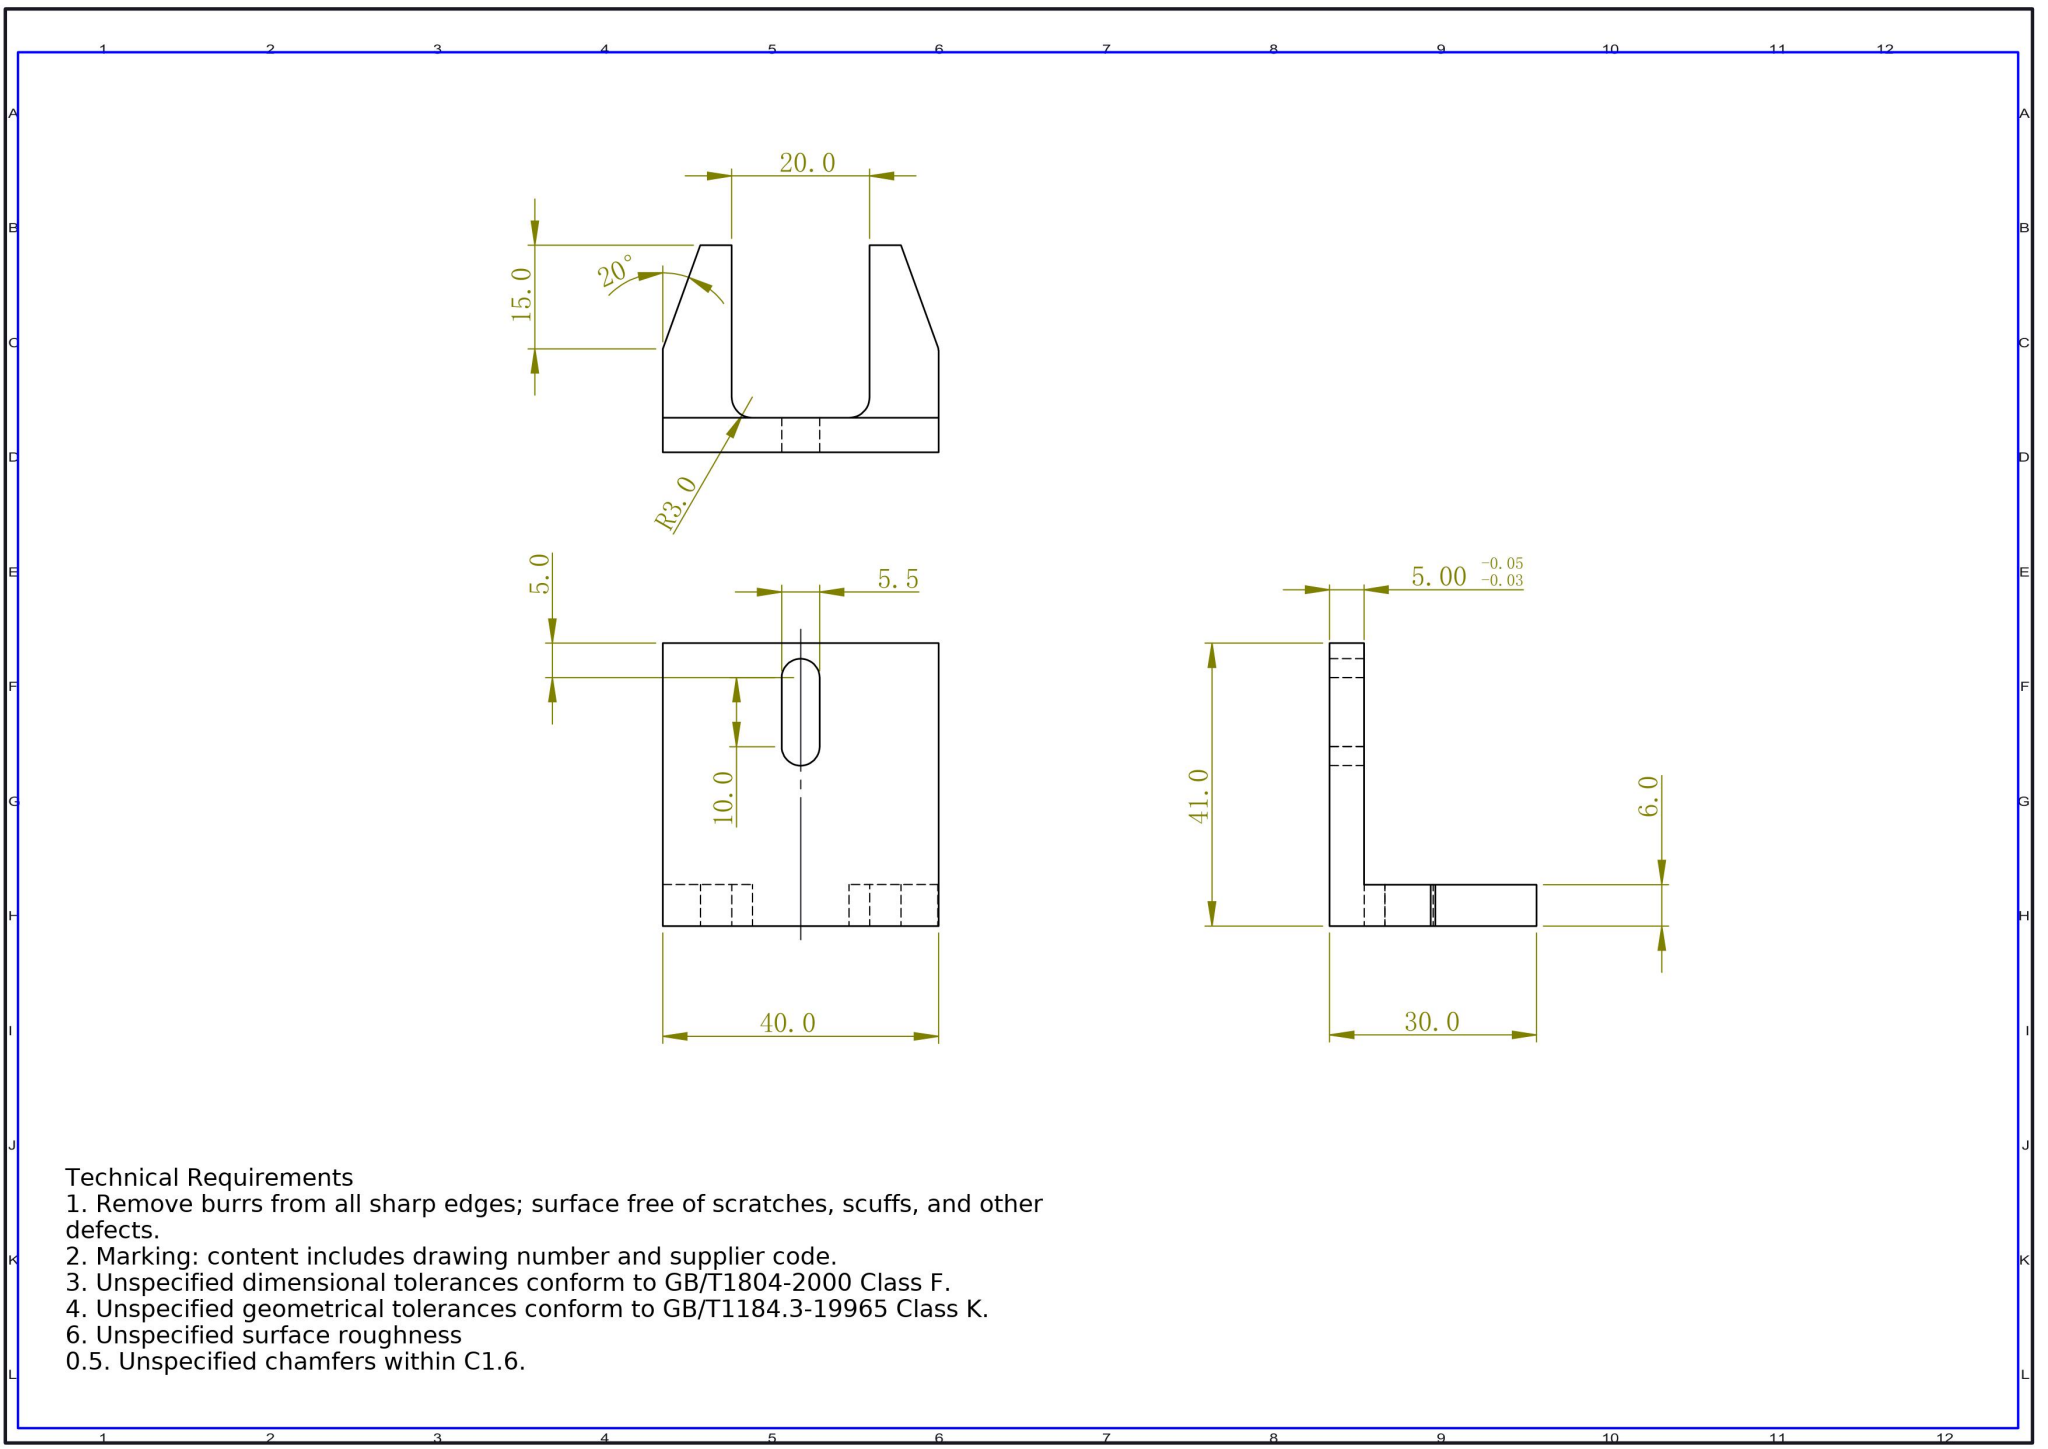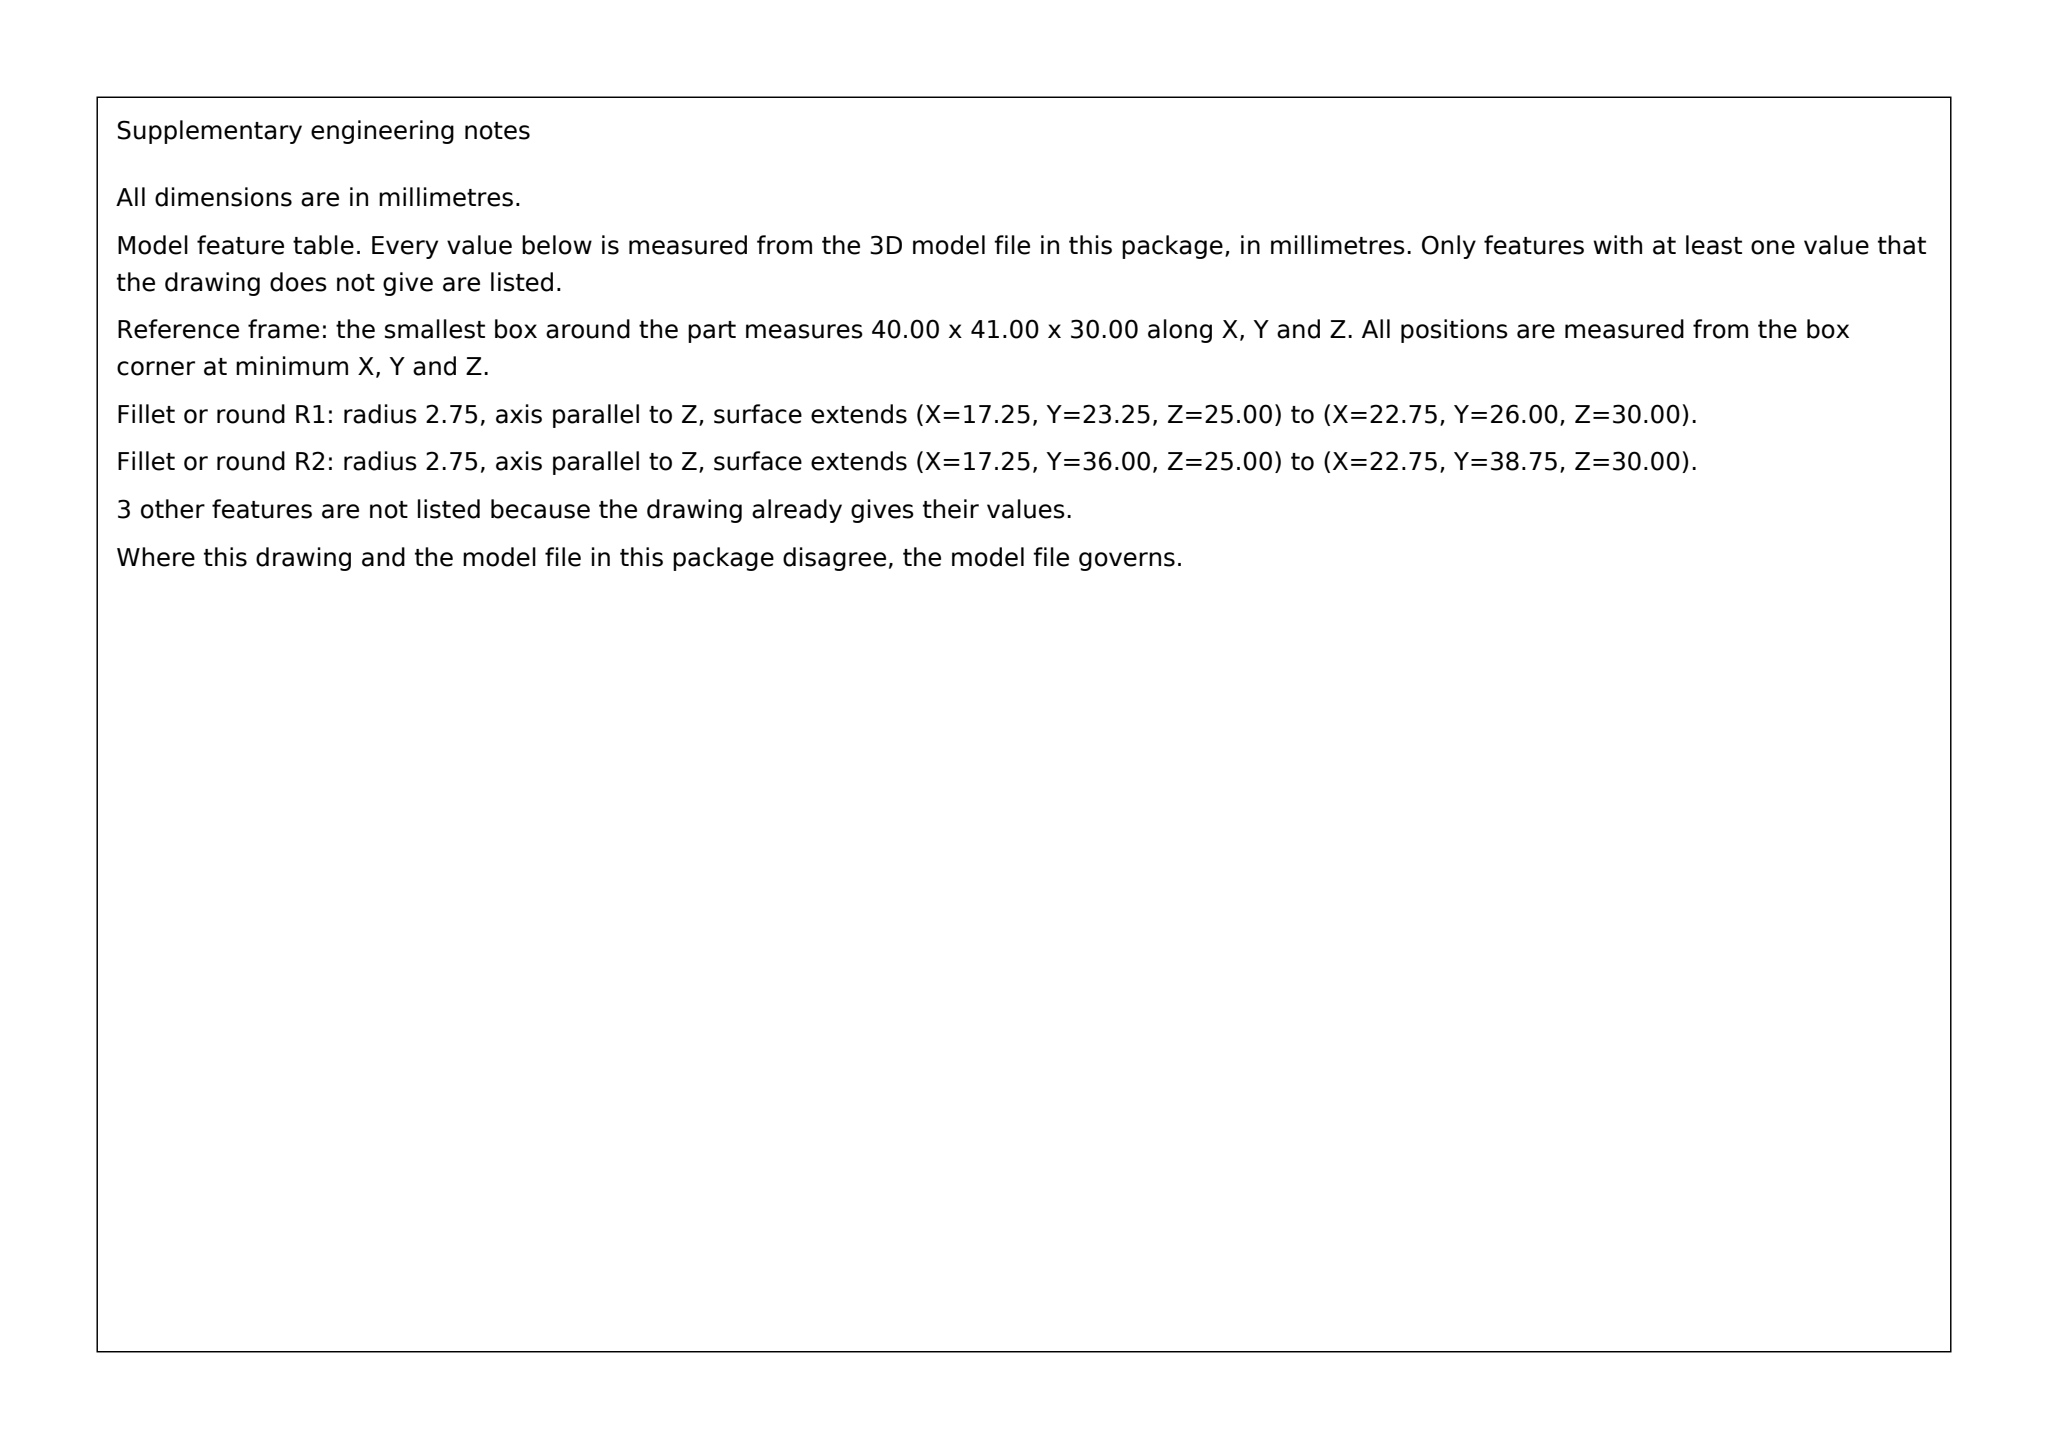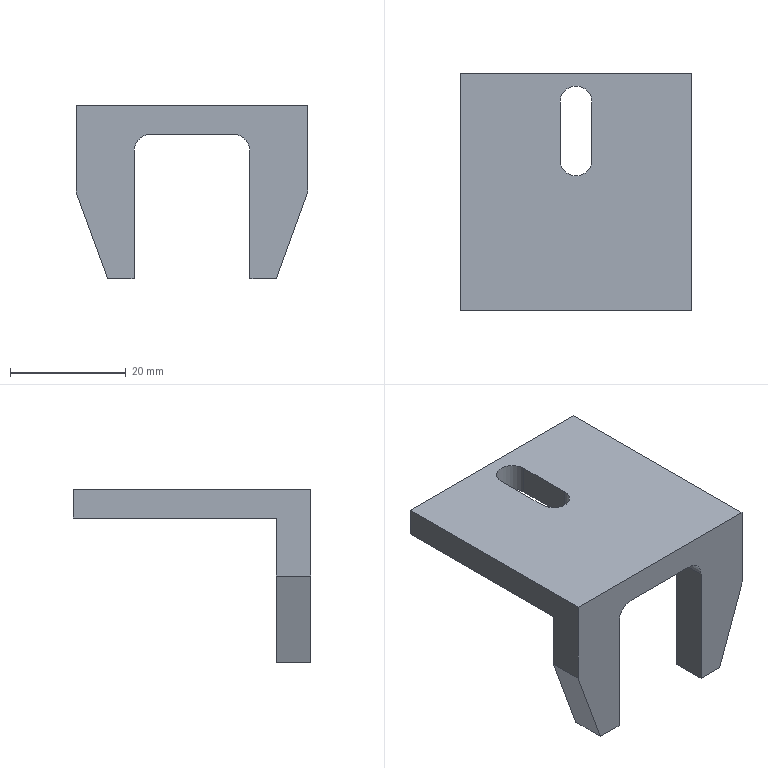Part | SolidWorks | mm | 1 solid | 21 faces | box 40 x 41 x 30 mm | volume 10338 mm3 | plane 16 | cylinder 5 | commonest cylinder face diameters 5.5 x2 6 x2 4 x1
build123d program:
from build123d import *

# Parameters (mm, degrees)
SKETCH1_W           = 40
SKETCH1_H           = 41
BOSS_EXTRUDE1_DEPTH = 5
BOSS_EXTRUDE3_DEPTH = 6
CUT_EXTRUDE3_DEPTH  = 53.019
FILLET1_R           = 2
FILLET4_R           = 3


with BuildPart() as part:
    # Sketch1 → Boss-Extrude1 (new body)
    with BuildSketch(Plane.XY.offset(5)):
        with Locations((0, 20.5)):
            Rectangle(SKETCH1_W, SKETCH1_H)
    extrude(amount=-BOSS_EXTRUDE1_DEPTH)

    # Sketch4 → Boss-Extrude3 (add)
    with BuildSketch(Plane.XZ):
        Polygon((20, -10), (20, 0), (10, 0), (10, -25), (14.54, -25), align=None)
    boss_extrude3 = extrude(amount=-BOSS_EXTRUDE3_DEPTH)

    # Sketch7 → Cut-Extrude3 (cut, through all)
    with BuildSketch(Plane(origin=(0, 0, 0), x_dir=(-1, 0, 0), z_dir=(0, 0, -1))):
        with BuildLine():
            Line((-2.75, 36), (-2.75, 26))
            ThreePointArc((-2.75, 26), (0, 23.25), (2.75, 26))
            Line((2.75, 26), (2.75, 36))
            ThreePointArc((2.75, 36), (0, 38.75), (-2.75, 36))
        make_face()
    extrude(amount=-CUT_EXTRUDE3_DEPTH, mode=Mode.SUBTRACT)

    # Fillet1
    fillet1_edges = [part.edges().sort_by_distance(p)[0] for p in [
        (20, 3, -10),
    ]]
    fillet(fillet1_edges, radius=FILLET1_R)

    # Mirror1: Boss-Extrude3 across plane
    add(boss_extrude3.mirror(Plane(origin=(0, 0, 0), x_dir=(0, 0, 1), z_dir=(1, 0, 0))))

    # Fillet4
    fillet4_edges = [part.edges().sort_by_distance(p)[0] for p in [
        (10, 3, 0),
        (-10, 3, 0),
    ]]
    fillet(fillet4_edges, radius=FILLET4_R)


solid = part.part